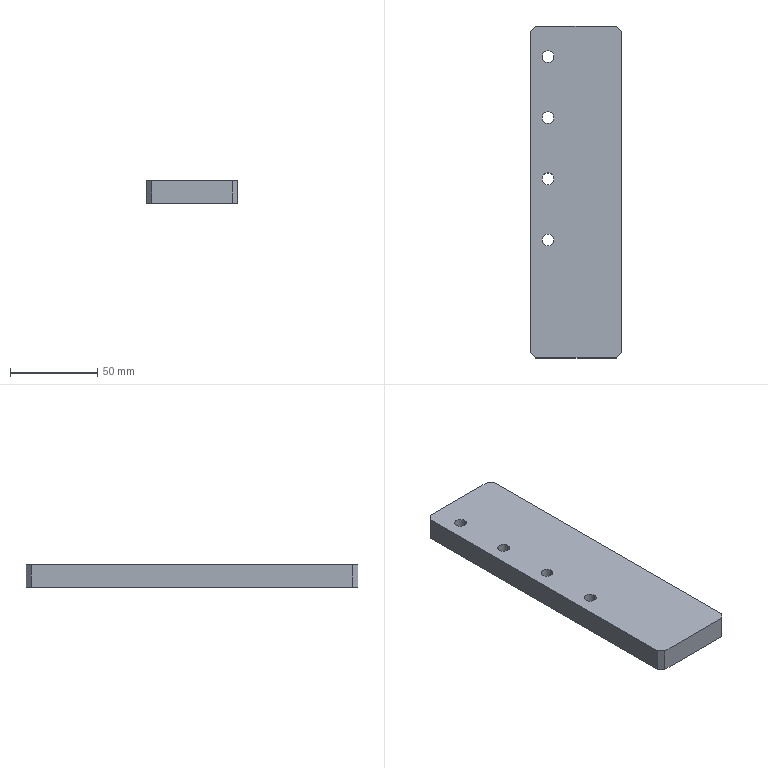Component | SolidWorks | STE21014.01-40-2 | 1 solid | 18 faces | box 52 x 190 x 13 mm | volume 126318 mm3 | plane 10 | cylinder 8 | commonest cylinder face diameters 6.8 x8 | material Q235
build123d program:
from build123d import *

# Parameters (mm, degrees)
SKETCH1_W           = 190
SKETCH1_H           = 52
BOSS_EXTRUDE1_DEPTH = 13
M8_TAPPED_HOLE1_D   = 6.8
CHAMFER1_SIZE       = 3


with BuildPart() as part:
    # Sketch1 → Boss-Extrude1 (new body)
    with BuildSketch(Plane(origin=(0, 0, 0), x_dir=(1, 0, 0), z_dir=(0, 1, 0))):
        Rectangle(SKETCH1_W, SKETCH1_H)
    extrude(amount=BOSS_EXTRUDE1_DEPTH)

    # M8 Tapped Hole1 (through all)
    with Locations(Plane(origin=(0, 13, 0), x_dir=(1, 0, 0), z_dir=(0, 1, 0))):
        with Locations((-27.5, -16), (7.5, -16), (42.5, -16), (77.5, -16)):
            Hole(M8_TAPPED_HOLE1_D / 2)

    # Chamfer1
    chamfer1_edges = [part.edges().sort_by_distance(p)[0] for p in [
        (-95, 6.5, -26),
        (95, 6.5, -26),
        (95, 6.5, 26),
        (-95, 6.5, 26),
    ]]
    chamfer(chamfer1_edges, length=CHAMFER1_SIZE)


solid = part.part

# Placed as in the assembly
solid = solid.moved(Location((616.25, 80, -610), (-90, -90, 0)))
STEP:
#1=COLOUR_RGB('',0.7922,0.8196,0.9333);
#2=FILL_AREA_STYLE_COLOUR('',#1);
#3=FILL_AREA_STYLE('',(#2));
#4=SURFACE_STYLE_FILL_AREA(#3);
#5=SURFACE_SIDE_STYLE('',(#4));
#6=SURFACE_STYLE_USAGE(.BOTH.,#5);
#7=PRESENTATION_STYLE_ASSIGNMENT((#6));
#8=CARTESIAN_POINT('',(23.766,2.067,-24.016));
#9=VERTEX_POINT('',#8);
#10=CARTESIAN_POINT('',(23.498,2.067,-24.016));
#11=VERTEX_POINT('',#10);
#12=CARTESIAN_POINT('',(23.632,2.067,-24.016));
#13=DIRECTION('',(-0.,-0.,-1.));
#14=DIRECTION('',(-1.,0.,0.));
#15=AXIS2_PLACEMENT_3D('',#12,#13,#14);
#16=CIRCLE('',#15,0.1339);
#17=EDGE_CURVE('',#9,#11,#16,.T.);
#18=ORIENTED_EDGE('',*,*,#17,.F.);
#19=CARTESIAN_POINT('',(23.766,2.067,-24.528));
#20=VERTEX_POINT('',#19);
#21=CARTESIAN_POINT('',(23.766,2.067,-24.528));
#22=DIRECTION('',(-0.,-0.,-1.));
#23=VECTOR('',#22,39.37);
#24=LINE('',#21,#23);
#25=EDGE_CURVE('',#9,#20,#24,.T.);
#26=ORIENTED_EDGE('',*,*,#25,.T.);
#27=CARTESIAN_POINT('',(23.498,2.067,-24.528));
#28=VERTEX_POINT('',#27);
#29=CARTESIAN_POINT('',(23.632,2.067,-24.528));
#30=DIRECTION('',(-0.,-0.,-1.));
#31=DIRECTION('',(-1.,0.,0.));
#32=AXIS2_PLACEMENT_3D('',#29,#30,#31);
#33=CIRCLE('',#32,0.1339);
#34=EDGE_CURVE('',#20,#28,#33,.T.);
#35=ORIENTED_EDGE('',*,*,#34,.T.);
#36=CARTESIAN_POINT('',(23.498,2.067,-24.528));
#37=DIRECTION('',(-0.,-0.,-1.));
#38=VECTOR('',#37,39.37);
#39=LINE('',#36,#38);
#40=EDGE_CURVE('',#11,#28,#39,.T.);
#41=ORIENTED_EDGE('',*,*,#40,.F.);
#42=EDGE_LOOP('',(#18,#26,#35,#41));
#43=FACE_OUTER_BOUND('',#42,.T.);
#44=CARTESIAN_POINT('',(23.632,2.067,-24.528));
#45=DIRECTION('',(-0.,-0.,-1.));
#46=DIRECTION('',(-1.,0.,0.));
#47=AXIS2_PLACEMENT_3D('',#44,#45,#46);
#48=CYLINDRICAL_SURFACE('',#47,0.1339);
#49=ADVANCED_FACE('',(#43),#48,.F.);
#50=CARTESIAN_POINT('',(23.766,3.445,-24.016));
#51=VERTEX_POINT('',#50);
#52=CARTESIAN_POINT('',(23.498,3.445,-24.016));
#53=VERTEX_POINT('',#52);
#54=CARTESIAN_POINT('',(23.632,3.445,-24.016));
#55=DIRECTION('',(-0.,-0.,-1.));
#56=DIRECTION('',(-1.,0.,0.));
#57=AXIS2_PLACEMENT_3D('',#54,#55,#56);
#58=CIRCLE('',#57,0.1339);
#59=EDGE_CURVE('',#51,#53,#58,.T.);
#60=ORIENTED_EDGE('',*,*,#59,.F.);
#61=CARTESIAN_POINT('',(23.766,3.445,-24.528));
#62=VERTEX_POINT('',#61);
#63=CARTESIAN_POINT('',(23.766,3.445,-24.528));
#64=DIRECTION('',(-0.,-0.,-1.));
#65=VECTOR('',#64,39.37);
#66=LINE('',#63,#65);
#67=EDGE_CURVE('',#51,#62,#66,.T.);
#68=ORIENTED_EDGE('',*,*,#67,.T.);
#69=CARTESIAN_POINT('',(23.498,3.445,-24.528));
#70=VERTEX_POINT('',#69);
#71=CARTESIAN_POINT('',(23.632,3.445,-24.528));
#72=DIRECTION('',(-0.,-0.,-1.));
#73=DIRECTION('',(-1.,0.,0.));
#74=AXIS2_PLACEMENT_3D('',#71,#72,#73);
#75=CIRCLE('',#74,0.1339);
#76=EDGE_CURVE('',#62,#70,#75,.T.);
#77=ORIENTED_EDGE('',*,*,#76,.T.);
#78=CARTESIAN_POINT('',(23.498,3.445,-24.528));
#79=DIRECTION('',(-0.,-0.,-1.));
#80=VECTOR('',#79,39.37);
#81=LINE('',#78,#80);
#82=EDGE_CURVE('',#53,#70,#81,.T.);
#83=ORIENTED_EDGE('',*,*,#82,.F.);
#84=EDGE_LOOP('',(#60,#68,#77,#83));
#85=FACE_OUTER_BOUND('',#84,.T.);
#86=CARTESIAN_POINT('',(23.632,3.445,-24.528));
#87=DIRECTION('',(-0.,-0.,-1.));
#88=DIRECTION('',(-1.,0.,0.));
#89=AXIS2_PLACEMENT_3D('',#86,#87,#88);
#90=CYLINDRICAL_SURFACE('',#89,0.1339);
#91=ADVANCED_FACE('',(#85),#90,.F.);
#92=CARTESIAN_POINT('',(23.766,4.823,-24.016));
#93=VERTEX_POINT('',#92);
#94=CARTESIAN_POINT('',(23.498,4.823,-24.016));
#95=VERTEX_POINT('',#94);
#96=CARTESIAN_POINT('',(23.632,4.823,-24.016));
#97=DIRECTION('',(-0.,-0.,-1.));
#98=DIRECTION('',(-1.,0.,0.));
#99=AXIS2_PLACEMENT_3D('',#96,#97,#98);
#100=CIRCLE('',#99,0.1339);
#101=EDGE_CURVE('',#93,#95,#100,.T.);
#102=ORIENTED_EDGE('',*,*,#101,.F.);
#103=CARTESIAN_POINT('',(23.766,4.823,-24.528));
#104=VERTEX_POINT('',#103);
#105=CARTESIAN_POINT('',(23.766,4.823,-24.528));
#106=DIRECTION('',(-0.,-0.,-1.));
#107=VECTOR('',#106,39.37);
#108=LINE('',#105,#107);
#109=EDGE_CURVE('',#93,#104,#108,.T.);
#110=ORIENTED_EDGE('',*,*,#109,.T.);
#111=CARTESIAN_POINT('',(23.498,4.823,-24.528));
#112=VERTEX_POINT('',#111);
#113=CARTESIAN_POINT('',(23.632,4.823,-24.528));
#114=DIRECTION('',(-0.,-0.,-1.));
#115=DIRECTION('',(-1.,0.,0.));
#116=AXIS2_PLACEMENT_3D('',#113,#114,#115);
#117=CIRCLE('',#116,0.1339);
#118=EDGE_CURVE('',#104,#112,#117,.T.);
#119=ORIENTED_EDGE('',*,*,#118,.T.);
#120=CARTESIAN_POINT('',(23.498,4.823,-24.528));
#121=DIRECTION('',(-0.,-0.,-1.));
#122=VECTOR('',#121,39.37);
#123=LINE('',#120,#122);
#124=EDGE_CURVE('',#95,#112,#123,.T.);
#125=ORIENTED_EDGE('',*,*,#124,.F.);
#126=EDGE_LOOP('',(#102,#110,#119,#125));
#127=FACE_OUTER_BOUND('',#126,.T.);
#128=CARTESIAN_POINT('',(23.632,4.823,-24.528));
#129=DIRECTION('',(-0.,-0.,-1.));
#130=DIRECTION('',(-1.,0.,0.));
#131=AXIS2_PLACEMENT_3D('',#128,#129,#130);
#132=CYLINDRICAL_SURFACE('',#131,0.1339);
#133=ADVANCED_FACE('',(#127),#132,.F.);
#134=CARTESIAN_POINT('',(23.766,6.201,-24.016));
#135=VERTEX_POINT('',#134);
#136=CARTESIAN_POINT('',(23.498,6.201,-24.016));
#137=VERTEX_POINT('',#136);
#138=CARTESIAN_POINT('',(23.632,6.201,-24.016));
#139=DIRECTION('',(-0.,-0.,-1.));
#140=DIRECTION('',(-1.,0.,0.));
#141=AXIS2_PLACEMENT_3D('',#138,#139,#140);
#142=CIRCLE('',#141,0.1339);
#143=EDGE_CURVE('',#135,#137,#142,.T.);
#144=ORIENTED_EDGE('',*,*,#143,.F.);
#145=CARTESIAN_POINT('',(23.766,6.201,-24.528));
#146=VERTEX_POINT('',#145);
#147=CARTESIAN_POINT('',(23.766,6.201,-24.528));
#148=DIRECTION('',(-0.,-0.,-1.));
#149=VECTOR('',#148,39.37);
#150=LINE('',#147,#149);
#151=EDGE_CURVE('',#135,#146,#150,.T.);
#152=ORIENTED_EDGE('',*,*,#151,.T.);
#153=CARTESIAN_POINT('',(23.498,6.201,-24.528));
#154=VERTEX_POINT('',#153);
#155=CARTESIAN_POINT('',(23.632,6.201,-24.528));
#156=DIRECTION('',(-0.,-0.,-1.));
#157=DIRECTION('',(-1.,0.,0.));
#158=AXIS2_PLACEMENT_3D('',#155,#156,#157);
#159=CIRCLE('',#158,0.1339);
#160=EDGE_CURVE('',#146,#154,#159,.T.);
#161=ORIENTED_EDGE('',*,*,#160,.T.);
#162=CARTESIAN_POINT('',(23.498,6.201,-24.528));
#163=DIRECTION('',(-0.,-0.,-1.));
#164=VECTOR('',#163,39.37);
#165=LINE('',#162,#164);
#166=EDGE_CURVE('',#137,#154,#165,.T.);
#167=ORIENTED_EDGE('',*,*,#166,.F.);
#168=EDGE_LOOP('',(#144,#152,#161,#167));
#169=FACE_OUTER_BOUND('',#168,.T.);
#170=CARTESIAN_POINT('',(23.632,6.201,-24.528));
#171=DIRECTION('',(-0.,-0.,-1.));
#172=DIRECTION('',(-1.,0.,0.));
#173=AXIS2_PLACEMENT_3D('',#170,#171,#172);
#174=CYLINDRICAL_SURFACE('',#173,0.1339);
#175=ADVANCED_FACE('',(#169),#174,.F.);
#176=CARTESIAN_POINT('',(25.167,-0.5906,-24.528));
#177=VERTEX_POINT('',#176);
#178=CARTESIAN_POINT('',(23.356,-0.5906,-24.528));
#179=VERTEX_POINT('',#178);
#180=CARTESIAN_POINT('',(23.238,-0.5906,-24.528));
#181=DIRECTION('',(-1.,0.,0.));
#182=VECTOR('',#181,39.37);
#183=LINE('',#180,#182);
#184=EDGE_CURVE('',#177,#179,#183,.T.);
#185=ORIENTED_EDGE('',*,*,#184,.F.);
#186=CARTESIAN_POINT('',(25.167,-0.5906,-24.016));
#187=VERTEX_POINT('',#186);
#188=CARTESIAN_POINT('',(25.167,-0.5906,-24.528));
#189=DIRECTION('',(0.,0.,1.));
#190=VECTOR('',#189,39.37);
#191=LINE('',#188,#190);
#192=EDGE_CURVE('',#177,#187,#191,.T.);
#193=ORIENTED_EDGE('',*,*,#192,.T.);
#194=CARTESIAN_POINT('',(23.356,-0.5906,-24.016));
#195=VERTEX_POINT('',#194);
#196=CARTESIAN_POINT('',(23.238,-0.5906,-24.016));
#197=DIRECTION('',(-1.,0.,0.));
#198=VECTOR('',#197,39.37);
#199=LINE('',#196,#198);
#200=EDGE_CURVE('',#187,#195,#199,.T.);
#201=ORIENTED_EDGE('',*,*,#200,.T.);
#202=CARTESIAN_POINT('',(23.356,-0.5906,-24.528));
#203=DIRECTION('',(-0.,-0.,-1.));
#204=VECTOR('',#203,39.37);
#205=LINE('',#202,#204);
#206=EDGE_CURVE('',#195,#179,#205,.T.);
#207=ORIENTED_EDGE('',*,*,#206,.T.);
#208=EDGE_LOOP('',(#185,#193,#201,#207));
#209=FACE_OUTER_BOUND('',#208,.T.);
#210=CARTESIAN_POINT('',(23.238,-0.5906,-24.528));
#211=DIRECTION('',(0.,1.,-0.));
#212=DIRECTION('',(1.,-0.,-0.));
#213=AXIS2_PLACEMENT_3D('',#210,#211,#212);
#214=PLANE('',#213);
#215=ADVANCED_FACE('',(#209),#214,.F.);
#216=CARTESIAN_POINT('',(23.238,-0.4724,-24.016));
#217=VERTEX_POINT('',#216);
#218=CARTESIAN_POINT('',(23.238,6.772,-24.016));
#219=VERTEX_POINT('',#218);
#220=CARTESIAN_POINT('',(23.238,6.89,-24.016));
#221=DIRECTION('',(0.,1.,-0.));
#222=VECTOR('',#221,39.37);
#223=LINE('',#220,#222);
#224=EDGE_CURVE('',#217,#219,#223,.T.);
#225=ORIENTED_EDGE('',*,*,#224,.T.);
#226=CARTESIAN_POINT('',(23.238,6.772,-24.528));
#227=VERTEX_POINT('',#226);
#228=CARTESIAN_POINT('',(23.238,6.772,-24.528));
#229=DIRECTION('',(-0.,-0.,-1.));
#230=VECTOR('',#229,39.37);
#231=LINE('',#228,#230);
#232=EDGE_CURVE('',#219,#227,#231,.T.);
#233=ORIENTED_EDGE('',*,*,#232,.T.);
#234=CARTESIAN_POINT('',(23.238,-0.4724,-24.528));
#235=VERTEX_POINT('',#234);
#236=CARTESIAN_POINT('',(23.238,6.89,-24.528));
#237=DIRECTION('',(0.,1.,-0.));
#238=VECTOR('',#237,39.37);
#239=LINE('',#236,#238);
#240=EDGE_CURVE('',#235,#227,#239,.T.);
#241=ORIENTED_EDGE('',*,*,#240,.F.);
#242=CARTESIAN_POINT('',(23.238,-0.4724,-24.528));
#243=DIRECTION('',(0.,0.,1.));
#244=VECTOR('',#243,39.37);
#245=LINE('',#242,#244);
#246=EDGE_CURVE('',#235,#217,#245,.T.);
#247=ORIENTED_EDGE('',*,*,#246,.T.);
#248=EDGE_LOOP('',(#225,#233,#241,#247));
#249=FACE_OUTER_BOUND('',#248,.T.);
#250=CARTESIAN_POINT('',(23.238,6.89,-24.528));
#251=DIRECTION('',(1.,-0.,-0.));
#252=DIRECTION('',(-0.,-1.,0.));
#253=AXIS2_PLACEMENT_3D('',#250,#251,#252);
#254=PLANE('',#253);
#255=ADVANCED_FACE('',(#249),#254,.F.);
#256=CARTESIAN_POINT('',(23.356,6.89,-24.528));
#257=VERTEX_POINT('',#256);
#258=CARTESIAN_POINT('',(25.167,6.89,-24.528));
#259=VERTEX_POINT('',#258);
#260=CARTESIAN_POINT('',(23.238,6.89,-24.528));
#261=DIRECTION('',(1.,-0.,-0.));
#262=VECTOR('',#261,39.37);
#263=LINE('',#260,#262);
#264=EDGE_CURVE('',#257,#259,#263,.T.);
#265=ORIENTED_EDGE('',*,*,#264,.F.);
#266=CARTESIAN_POINT('',(23.356,6.89,-24.016));
#267=VERTEX_POINT('',#266);
#268=CARTESIAN_POINT('',(23.356,6.89,-24.528));
#269=DIRECTION('',(0.,0.,1.));
#270=VECTOR('',#269,39.37);
#271=LINE('',#268,#270);
#272=EDGE_CURVE('',#257,#267,#271,.T.);
#273=ORIENTED_EDGE('',*,*,#272,.T.);
#274=CARTESIAN_POINT('',(25.167,6.89,-24.016));
#275=VERTEX_POINT('',#274);
#276=CARTESIAN_POINT('',(23.238,6.89,-24.016));
#277=DIRECTION('',(1.,-0.,-0.));
#278=VECTOR('',#277,39.37);
#279=LINE('',#276,#278);
#280=EDGE_CURVE('',#267,#275,#279,.T.);
#281=ORIENTED_EDGE('',*,*,#280,.T.);
#282=CARTESIAN_POINT('',(25.167,6.89,-24.528));
#283=DIRECTION('',(-0.,-0.,-1.));
#284=VECTOR('',#283,39.37);
#285=LINE('',#282,#284);
#286=EDGE_CURVE('',#275,#259,#285,.T.);
#287=ORIENTED_EDGE('',*,*,#286,.T.);
#288=EDGE_LOOP('',(#265,#273,#281,#287));
#289=FACE_OUTER_BOUND('',#288,.T.);
#290=CARTESIAN_POINT('',(23.238,6.89,-24.528));
#291=DIRECTION('',(-0.,-1.,0.));
#292=DIRECTION('',(-1.,0.,0.));
#293=AXIS2_PLACEMENT_3D('',#290,#291,#292);
#294=PLANE('',#293);
#295=ADVANCED_FACE('',(#289),#294,.F.);
#296=CARTESIAN_POINT('',(25.285,6.772,-24.528));
#297=VERTEX_POINT('',#296);
#298=CARTESIAN_POINT('',(25.285,-0.4724,-24.528));
#299=VERTEX_POINT('',#298);
#300=CARTESIAN_POINT('',(25.285,6.89,-24.528));
#301=DIRECTION('',(-0.,-1.,0.));
#302=VECTOR('',#301,39.37);
#303=LINE('',#300,#302);
#304=EDGE_CURVE('',#297,#299,#303,.T.);
#305=ORIENTED_EDGE('',*,*,#304,.F.);
#306=CARTESIAN_POINT('',(25.285,6.772,-24.016));
#307=VERTEX_POINT('',#306);
#308=CARTESIAN_POINT('',(25.285,6.772,-24.528));
#309=DIRECTION('',(0.,0.,1.));
#310=VECTOR('',#309,39.37);
#311=LINE('',#308,#310);
#312=EDGE_CURVE('',#297,#307,#311,.T.);
#313=ORIENTED_EDGE('',*,*,#312,.T.);
#314=CARTESIAN_POINT('',(25.285,-0.4724,-24.016));
#315=VERTEX_POINT('',#314);
#316=CARTESIAN_POINT('',(25.285,6.89,-24.016));
#317=DIRECTION('',(-0.,-1.,0.));
#318=VECTOR('',#317,39.37);
#319=LINE('',#316,#318);
#320=EDGE_CURVE('',#307,#315,#319,.T.);
#321=ORIENTED_EDGE('',*,*,#320,.T.);
#322=CARTESIAN_POINT('',(25.285,-0.4724,-24.528));
#323=DIRECTION('',(-0.,-0.,-1.));
#324=VECTOR('',#323,39.37);
#325=LINE('',#322,#324);
#326=EDGE_CURVE('',#315,#299,#325,.T.);
#327=ORIENTED_EDGE('',*,*,#326,.T.);
#328=EDGE_LOOP('',(#305,#313,#321,#327));
#329=FACE_OUTER_BOUND('',#328,.T.);
#330=CARTESIAN_POINT('',(25.285,6.89,-24.528));
#331=DIRECTION('',(-1.,0.,0.));
#332=DIRECTION('',(0.,1.,-0.));
#333=AXIS2_PLACEMENT_3D('',#330,#331,#332);
#334=PLANE('',#333);
#335=ADVANCED_FACE('',(#329),#334,.F.);
#336=CARTESIAN_POINT('',(23.632,2.067,-24.528));
#337=DIRECTION('',(-0.,-0.,-1.));
#338=DIRECTION('',(-1.,0.,0.));
#339=AXIS2_PLACEMENT_3D('',#336,#337,#338);
#340=CIRCLE('',#339,0.1339);
#341=EDGE_CURVE('',#28,#20,#340,.T.);
#342=ORIENTED_EDGE('',*,*,#341,.F.);
#343=ORIENTED_EDGE('',*,*,#34,.F.);
#344=EDGE_LOOP('',(#342,#343));
#345=FACE_BOUND('',#344,.T.);
#346=CARTESIAN_POINT('',(23.632,3.445,-24.528));
#347=DIRECTION('',(-0.,-0.,-1.));
#348=DIRECTION('',(-1.,0.,0.));
#349=AXIS2_PLACEMENT_3D('',#346,#347,#348);
#350=CIRCLE('',#349,0.1339);
#351=EDGE_CURVE('',#70,#62,#350,.T.);
#352=ORIENTED_EDGE('',*,*,#351,.F.);
#353=ORIENTED_EDGE('',*,*,#76,.F.);
#354=EDGE_LOOP('',(#352,#353));
#355=FACE_BOUND('',#354,.T.);
#356=CARTESIAN_POINT('',(23.632,4.823,-24.528));
#357=DIRECTION('',(-0.,-0.,-1.));
#358=DIRECTION('',(-1.,0.,0.));
#359=AXIS2_PLACEMENT_3D('',#356,#357,#358);
#360=CIRCLE('',#359,0.1339);
#361=EDGE_CURVE('',#112,#104,#360,.T.);
#362=ORIENTED_EDGE('',*,*,#361,.F.);
#363=ORIENTED_EDGE('',*,*,#118,.F.);
#364=EDGE_LOOP('',(#362,#363));
#365=FACE_BOUND('',#364,.T.);
#366=CARTESIAN_POINT('',(23.632,6.201,-24.528));
#367=DIRECTION('',(-0.,-0.,-1.));
#368=DIRECTION('',(-1.,0.,0.));
#369=AXIS2_PLACEMENT_3D('',#366,#367,#368);
#370=CIRCLE('',#369,0.1339);
#371=EDGE_CURVE('',#154,#146,#370,.T.);
#372=ORIENTED_EDGE('',*,*,#371,.F.);
#373=ORIENTED_EDGE('',*,*,#160,.F.);
#374=EDGE_LOOP('',(#372,#373));
#375=FACE_BOUND('',#374,.T.);
#376=ORIENTED_EDGE('',*,*,#240,.T.);
#377=CARTESIAN_POINT('',(21.939,5.472,-24.528));
#378=DIRECTION('',(0.7071,0.7071,-0.));
#379=VECTOR('',#378,39.37);
#380=LINE('',#377,#379);
#381=EDGE_CURVE('',#227,#257,#380,.T.);
#382=ORIENTED_EDGE('',*,*,#381,.T.);
#383=ORIENTED_EDGE('',*,*,#264,.T.);
#384=CARTESIAN_POINT('',(26.585,5.472,-24.528));
#385=DIRECTION('',(0.7071,-0.7071,0.));
#386=VECTOR('',#385,39.37);
#387=LINE('',#384,#386);
#388=EDGE_CURVE('',#259,#297,#387,.T.);
#389=ORIENTED_EDGE('',*,*,#388,.T.);
#390=ORIENTED_EDGE('',*,*,#304,.T.);
#391=CARTESIAN_POINT('',(26.585,0.8268,-24.528));
#392=DIRECTION('',(-0.7071,-0.7071,0.));
#393=VECTOR('',#392,39.37);
#394=LINE('',#391,#393);
#395=EDGE_CURVE('',#299,#177,#394,.T.);
#396=ORIENTED_EDGE('',*,*,#395,.T.);
#397=ORIENTED_EDGE('',*,*,#184,.T.);
#398=CARTESIAN_POINT('',(21.939,0.8268,-24.528));
#399=DIRECTION('',(-0.7071,0.7071,-0.));
#400=VECTOR('',#399,39.37);
#401=LINE('',#398,#400);
#402=EDGE_CURVE('',#179,#235,#401,.T.);
#403=ORIENTED_EDGE('',*,*,#402,.T.);
#404=EDGE_LOOP('',(#376,#382,#383,#389,#390,#396,#397,#403));
#405=FACE_OUTER_BOUND('',#404,.T.);
#406=CARTESIAN_POINT('',(24.262,3.15,-24.528));
#407=DIRECTION('',(-0.,-0.,-1.));
#408=DIRECTION('',(-1.,0.,0.));
#409=AXIS2_PLACEMENT_3D('',#406,#407,#408);
#410=PLANE('',#409);
#411=ADVANCED_FACE('',(#345,#355,#365,#375,#405),#410,.T.);
#412=CARTESIAN_POINT('',(23.632,2.067,-24.016));
#413=DIRECTION('',(-0.,-0.,-1.));
#414=DIRECTION('',(-1.,0.,0.));
#415=AXIS2_PLACEMENT_3D('',#412,#413,#414);
#416=CIRCLE('',#415,0.1339);
#417=EDGE_CURVE('',#11,#9,#416,.T.);
#418=ORIENTED_EDGE('',*,*,#417,.T.);
#419=ORIENTED_EDGE('',*,*,#17,.T.);
#420=EDGE_LOOP('',(#418,#419));
#421=FACE_BOUND('',#420,.T.);
#422=CARTESIAN_POINT('',(23.632,3.445,-24.016));
#423=DIRECTION('',(-0.,-0.,-1.));
#424=DIRECTION('',(-1.,0.,0.));
#425=AXIS2_PLACEMENT_3D('',#422,#423,#424);
#426=CIRCLE('',#425,0.1339);
#427=EDGE_CURVE('',#53,#51,#426,.T.);
#428=ORIENTED_EDGE('',*,*,#427,.T.);
#429=ORIENTED_EDGE('',*,*,#59,.T.);
#430=EDGE_LOOP('',(#428,#429));
#431=FACE_BOUND('',#430,.T.);
#432=CARTESIAN_POINT('',(23.632,4.823,-24.016));
#433=DIRECTION('',(-0.,-0.,-1.));
#434=DIRECTION('',(-1.,0.,0.));
#435=AXIS2_PLACEMENT_3D('',#432,#433,#434);
#436=CIRCLE('',#435,0.1339);
#437=EDGE_CURVE('',#95,#93,#436,.T.);
#438=ORIENTED_EDGE('',*,*,#437,.T.);
#439=ORIENTED_EDGE('',*,*,#101,.T.);
#440=EDGE_LOOP('',(#438,#439));
#441=FACE_BOUND('',#440,.T.);
#442=CARTESIAN_POINT('',(23.632,6.201,-24.016));
#443=DIRECTION('',(-0.,-0.,-1.));
#444=DIRECTION('',(-1.,0.,0.));
#445=AXIS2_PLACEMENT_3D('',#442,#443,#444);
#446=CIRCLE('',#445,0.1339);
#447=EDGE_CURVE('',#137,#135,#446,.T.);
#448=ORIENTED_EDGE('',*,*,#447,.T.);
#449=ORIENTED_EDGE('',*,*,#143,.T.);
#450=EDGE_LOOP('',(#448,#449));
#451=FACE_BOUND('',#450,.T.);
#452=ORIENTED_EDGE('',*,*,#280,.F.);
#453=CARTESIAN_POINT('',(23.356,6.89,-24.016));
#454=DIRECTION('',(-0.7071,-0.7071,0.));
#455=VECTOR('',#454,39.37);
#456=LINE('',#453,#455);
#457=EDGE_CURVE('',#267,#219,#456,.T.);
#458=ORIENTED_EDGE('',*,*,#457,.T.);
#459=ORIENTED_EDGE('',*,*,#224,.F.);
#460=CARTESIAN_POINT('',(23.238,-0.4724,-24.016));
#461=DIRECTION('',(0.7071,-0.7071,0.));
#462=VECTOR('',#461,39.37);
#463=LINE('',#460,#462);
#464=EDGE_CURVE('',#217,#195,#463,.T.);
#465=ORIENTED_EDGE('',*,*,#464,.T.);
#466=ORIENTED_EDGE('',*,*,#200,.F.);
#467=CARTESIAN_POINT('',(25.167,-0.5906,-24.016));
#468=DIRECTION('',(0.7071,0.7071,-0.));
#469=VECTOR('',#468,39.37);
#470=LINE('',#467,#469);
#471=EDGE_CURVE('',#187,#315,#470,.T.);
#472=ORIENTED_EDGE('',*,*,#471,.T.);
#473=ORIENTED_EDGE('',*,*,#320,.F.);
#474=CARTESIAN_POINT('',(25.285,6.772,-24.016));
#475=DIRECTION('',(-0.7071,0.7071,-0.));
#476=VECTOR('',#475,39.37);
#477=LINE('',#474,#476);
#478=EDGE_CURVE('',#307,#275,#477,.T.);
#479=ORIENTED_EDGE('',*,*,#478,.T.);
#480=EDGE_LOOP('',(#452,#458,#459,#465,#466,#472,#473,#479));
#481=FACE_OUTER_BOUND('',#480,.T.);
#482=CARTESIAN_POINT('',(24.262,3.15,-24.016));
#483=DIRECTION('',(-0.,-0.,-1.));
#484=DIRECTION('',(-1.,0.,0.));
#485=AXIS2_PLACEMENT_3D('',#482,#483,#484);
#486=PLANE('',#485);
#487=ADVANCED_FACE('',(#421,#431,#441,#451,#481),#486,.F.);
#488=ORIENTED_EDGE('',*,*,#151,.F.);
#489=ORIENTED_EDGE('',*,*,#447,.F.);
#490=ORIENTED_EDGE('',*,*,#166,.T.);
#491=ORIENTED_EDGE('',*,*,#371,.T.);
#492=EDGE_LOOP('',(#488,#489,#490,#491));
#493=FACE_OUTER_BOUND('',#492,.T.);
#494=CARTESIAN_POINT('',(23.632,6.201,-24.528));
#495=DIRECTION('',(-0.,-0.,-1.));
#496=DIRECTION('',(-1.,0.,0.));
#497=AXIS2_PLACEMENT_3D('',#494,#495,#496);
#498=CYLINDRICAL_SURFACE('',#497,0.1339);
#499=ADVANCED_FACE('',(#493),#498,.F.);
#500=ORIENTED_EDGE('',*,*,#109,.F.);
#501=ORIENTED_EDGE('',*,*,#437,.F.);
#502=ORIENTED_EDGE('',*,*,#124,.T.);
#503=ORIENTED_EDGE('',*,*,#361,.T.);
#504=EDGE_LOOP('',(#500,#501,#502,#503));
#505=FACE_OUTER_BOUND('',#504,.T.);
#506=CARTESIAN_POINT('',(23.632,4.823,-24.528));
#507=DIRECTION('',(-0.,-0.,-1.));
#508=DIRECTION('',(-1.,0.,0.));
#509=AXIS2_PLACEMENT_3D('',#506,#507,#508);
#510=CYLINDRICAL_SURFACE('',#509,0.1339);
#511=ADVANCED_FACE('',(#505),#510,.F.);
#512=ORIENTED_EDGE('',*,*,#67,.F.);
#513=ORIENTED_EDGE('',*,*,#427,.F.);
#514=ORIENTED_EDGE('',*,*,#82,.T.);
#515=ORIENTED_EDGE('',*,*,#351,.T.);
#516=EDGE_LOOP('',(#512,#513,#514,#515));
#517=FACE_OUTER_BOUND('',#516,.T.);
#518=CARTESIAN_POINT('',(23.632,3.445,-24.528));
#519=DIRECTION('',(-0.,-0.,-1.));
#520=DIRECTION('',(-1.,0.,0.));
#521=AXIS2_PLACEMENT_3D('',#518,#519,#520);
#522=CYLINDRICAL_SURFACE('',#521,0.1339);
#523=ADVANCED_FACE('',(#517),#522,.F.);
#524=ORIENTED_EDGE('',*,*,#25,.F.);
#525=ORIENTED_EDGE('',*,*,#417,.F.);
#526=ORIENTED_EDGE('',*,*,#40,.T.);
#527=ORIENTED_EDGE('',*,*,#341,.T.);
#528=EDGE_LOOP('',(#524,#525,#526,#527));
#529=FACE_OUTER_BOUND('',#528,.T.);
#530=CARTESIAN_POINT('',(23.632,2.067,-24.528));
#531=DIRECTION('',(-0.,-0.,-1.));
#532=DIRECTION('',(-1.,0.,0.));
#533=AXIS2_PLACEMENT_3D('',#530,#531,#532);
#534=CYLINDRICAL_SURFACE('',#533,0.1339);
#535=ADVANCED_FACE('',(#529),#534,.F.);
#536=ORIENTED_EDGE('',*,*,#381,.F.);
#537=ORIENTED_EDGE('',*,*,#232,.F.);
#538=ORIENTED_EDGE('',*,*,#457,.F.);
#539=ORIENTED_EDGE('',*,*,#272,.F.);
#540=EDGE_LOOP('',(#536,#537,#538,#539));
#541=FACE_OUTER_BOUND('',#540,.T.);
#542=CARTESIAN_POINT('',(23.356,6.89,-24.528));
#543=DIRECTION('',(0.7071,-0.7071,0.));
#544=DIRECTION('',(0.,0.,1.));
#545=AXIS2_PLACEMENT_3D('',#542,#543,#544);
#546=PLANE('',#545);
#547=ADVANCED_FACE('',(#541),#546,.F.);
#548=ORIENTED_EDGE('',*,*,#388,.F.);
#549=ORIENTED_EDGE('',*,*,#286,.F.);
#550=ORIENTED_EDGE('',*,*,#478,.F.);
#551=ORIENTED_EDGE('',*,*,#312,.F.);
#552=EDGE_LOOP('',(#548,#549,#550,#551));
#553=FACE_OUTER_BOUND('',#552,.T.);
#554=CARTESIAN_POINT('',(25.285,6.772,-24.528));
#555=DIRECTION('',(-0.7071,-0.7071,0.));
#556=DIRECTION('',(0.,0.,1.));
#557=AXIS2_PLACEMENT_3D('',#554,#555,#556);
#558=PLANE('',#557);
#559=ADVANCED_FACE('',(#553),#558,.F.);
#560=ORIENTED_EDGE('',*,*,#395,.F.);
#561=ORIENTED_EDGE('',*,*,#326,.F.);
#562=ORIENTED_EDGE('',*,*,#471,.F.);
#563=ORIENTED_EDGE('',*,*,#192,.F.);
#564=EDGE_LOOP('',(#560,#561,#562,#563));
#565=FACE_OUTER_BOUND('',#564,.T.);
#566=CARTESIAN_POINT('',(25.167,-0.5906,-24.528));
#567=DIRECTION('',(-0.7071,0.7071,-0.));
#568=DIRECTION('',(0.,0.,1.));
#569=AXIS2_PLACEMENT_3D('',#566,#567,#568);
#570=PLANE('',#569);
#571=ADVANCED_FACE('',(#565),#570,.F.);
#572=ORIENTED_EDGE('',*,*,#402,.F.);
#573=ORIENTED_EDGE('',*,*,#206,.F.);
#574=ORIENTED_EDGE('',*,*,#464,.F.);
#575=ORIENTED_EDGE('',*,*,#246,.F.);
#576=EDGE_LOOP('',(#572,#573,#574,#575));
#577=FACE_OUTER_BOUND('',#576,.T.);
#578=CARTESIAN_POINT('',(23.238,-0.4724,-24.528));
#579=DIRECTION('',(0.7071,0.7071,-0.));
#580=DIRECTION('',(0.,0.,1.));
#581=AXIS2_PLACEMENT_3D('',#578,#579,#580);
#582=PLANE('',#581);
#583=ADVANCED_FACE('',(#577),#582,.F.);
#584=CLOSED_SHELL('',(#49,#91,#133,#175,#215,#255,#295,#335,#411,#487,#499,#511,#523,#535,#547,#559,#571,#583));
#585=MANIFOLD_SOLID_BREP('',#584);
#586=STYLED_ITEM('',(#7),#585);
#587=(LENGTH_UNIT()NAMED_UNIT(*)SI_UNIT($,.METRE.));
#588=LENGTH_MEASURE_WITH_UNIT(LENGTH_MEASURE(0.0254),#587);
#589=DIMENSIONAL_EXPONENTS(1.,0.,0.,0.,0.,0.,0.);
#590=(CONVERSION_BASED_UNIT('',#588)LENGTH_UNIT()NAMED_UNIT(#589));
#591=UNCERTAINTY_MEASURE_WITH_UNIT(LENGTH_MEASURE(0.00001),#590,'','');
#592=(NAMED_UNIT(*)PLANE_ANGLE_UNIT()SI_UNIT($,.RADIAN.));
#593=(NAMED_UNIT(*)SI_UNIT($,.STERADIAN.)SOLID_ANGLE_UNIT());
#594=(GEOMETRIC_REPRESENTATION_CONTEXT(3)GLOBAL_UNCERTAINTY_ASSIGNED_CONTEXT((#591))GLOBAL_UNIT_ASSIGNED_CONTEXT((#590,#592,#593))REPRESENTATION_CONTEXT('',''));
#595=MECHANICAL_DESIGN_GEOMETRIC_PRESENTATION_REPRESENTATION('',(#586),#594);
#596=CARTESIAN_POINT('',(0.,0.,0.));
#597=DIRECTION('',(0.,0.,1.));
#598=DIRECTION('',(1.,0.,0.));
#599=AXIS2_PLACEMENT_3D('',#596,#597,#598);
#600=(LENGTH_UNIT()NAMED_UNIT(*)SI_UNIT($,.METRE.));
#601=LENGTH_MEASURE_WITH_UNIT(LENGTH_MEASURE(0.0254),#600);
#602=DIMENSIONAL_EXPONENTS(1.,0.,0.,0.,0.,0.,0.);
#603=(CONVERSION_BASED_UNIT('',#601)LENGTH_UNIT()NAMED_UNIT(#602));
#604=UNCERTAINTY_MEASURE_WITH_UNIT(LENGTH_MEASURE(0.00001),#603,'','');
#605=(NAMED_UNIT(*)PLANE_ANGLE_UNIT()SI_UNIT($,.RADIAN.));
#606=(NAMED_UNIT(*)SI_UNIT($,.STERADIAN.)SOLID_ANGLE_UNIT());
#607=(GEOMETRIC_REPRESENTATION_CONTEXT(3)GLOBAL_UNCERTAINTY_ASSIGNED_CONTEXT((#604))GLOBAL_UNIT_ASSIGNED_CONTEXT((#603,#605,#606))REPRESENTATION_CONTEXT('',''));
#608=ADVANCED_BREP_SHAPE_REPRESENTATION('',(#585,#599),#607);
#609=PRESENTATION_LAYER_ASSIGNMENT('','',(#586));